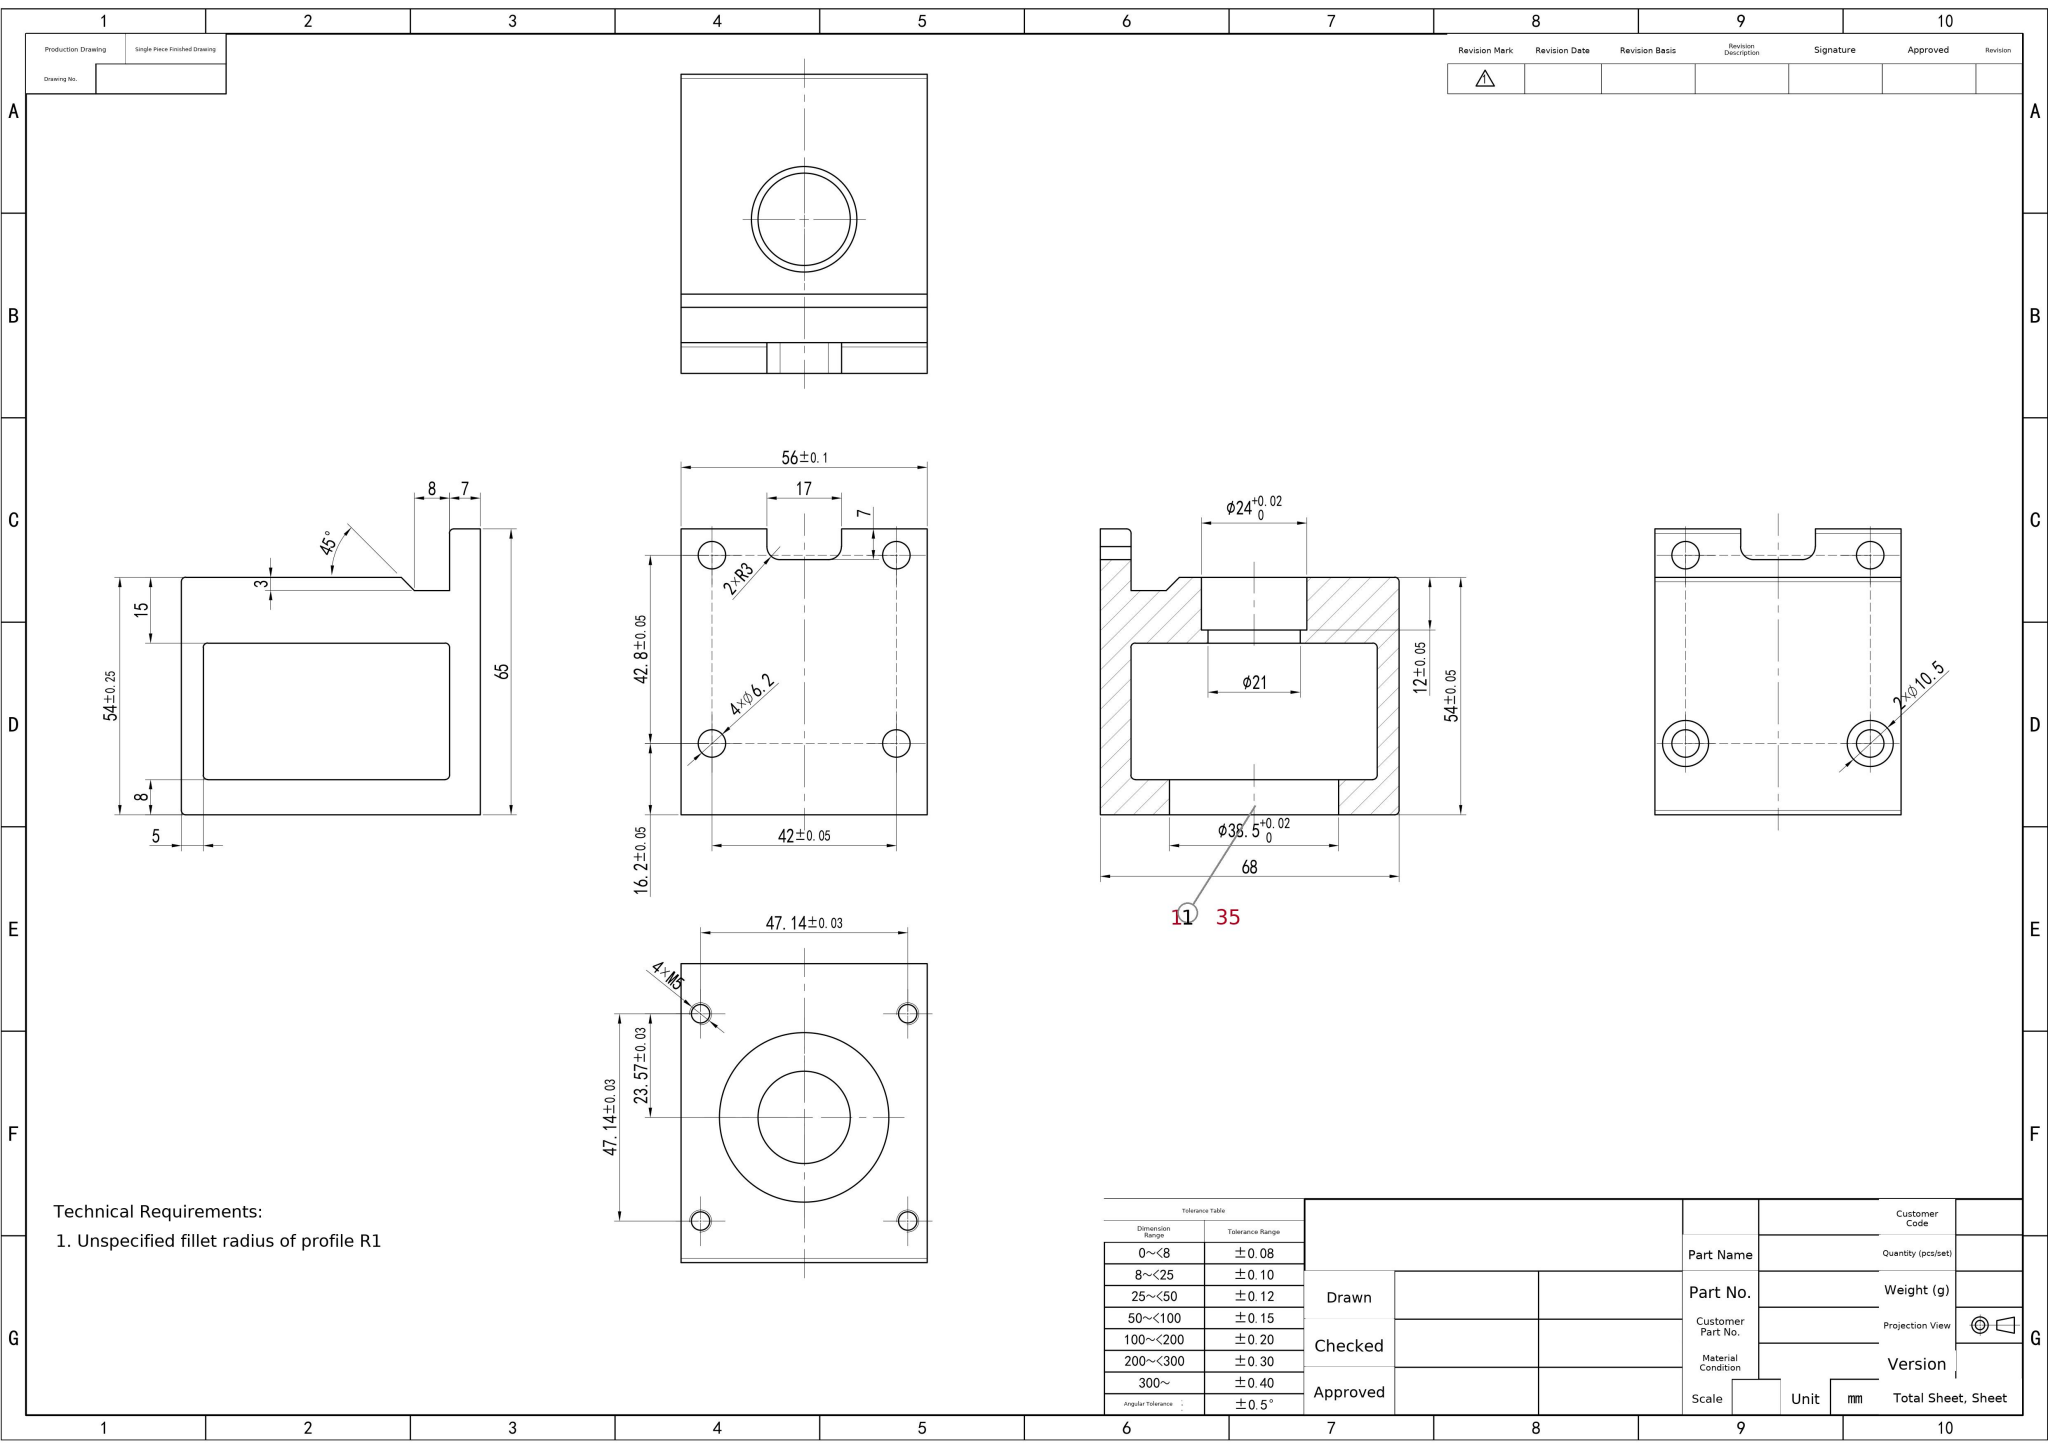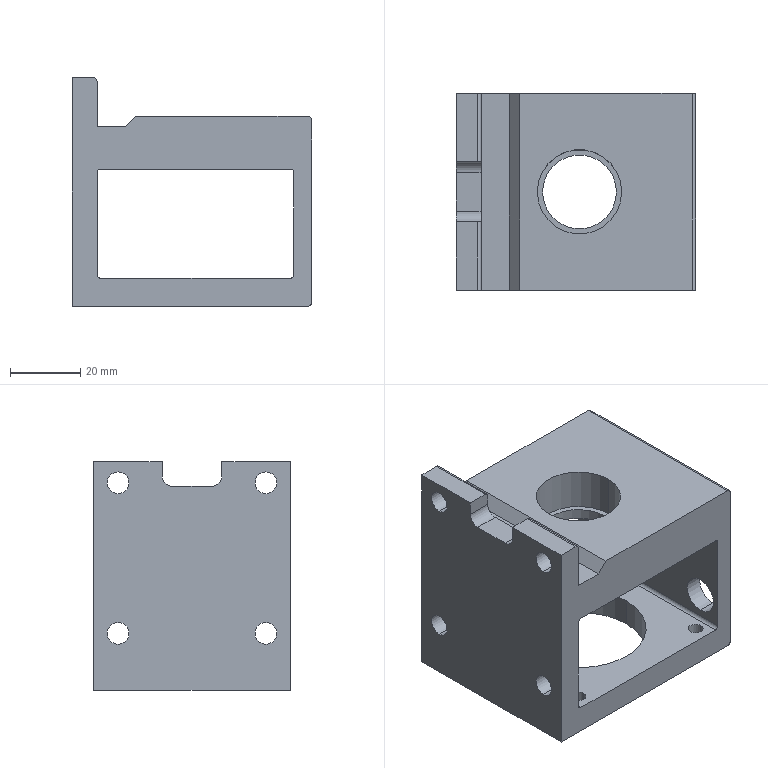Part | SolidWorks | mm | 1 solid | 55 faces | box 68 x 56 x 65 mm | volume 92406 mm3 | cylinder 36 | plane 19 | commonest cylinder face diameters 6.2 x8 4.2 x8 2 x8 10.5 x4 38.5 x2 21 x2 24 x2 6 x2